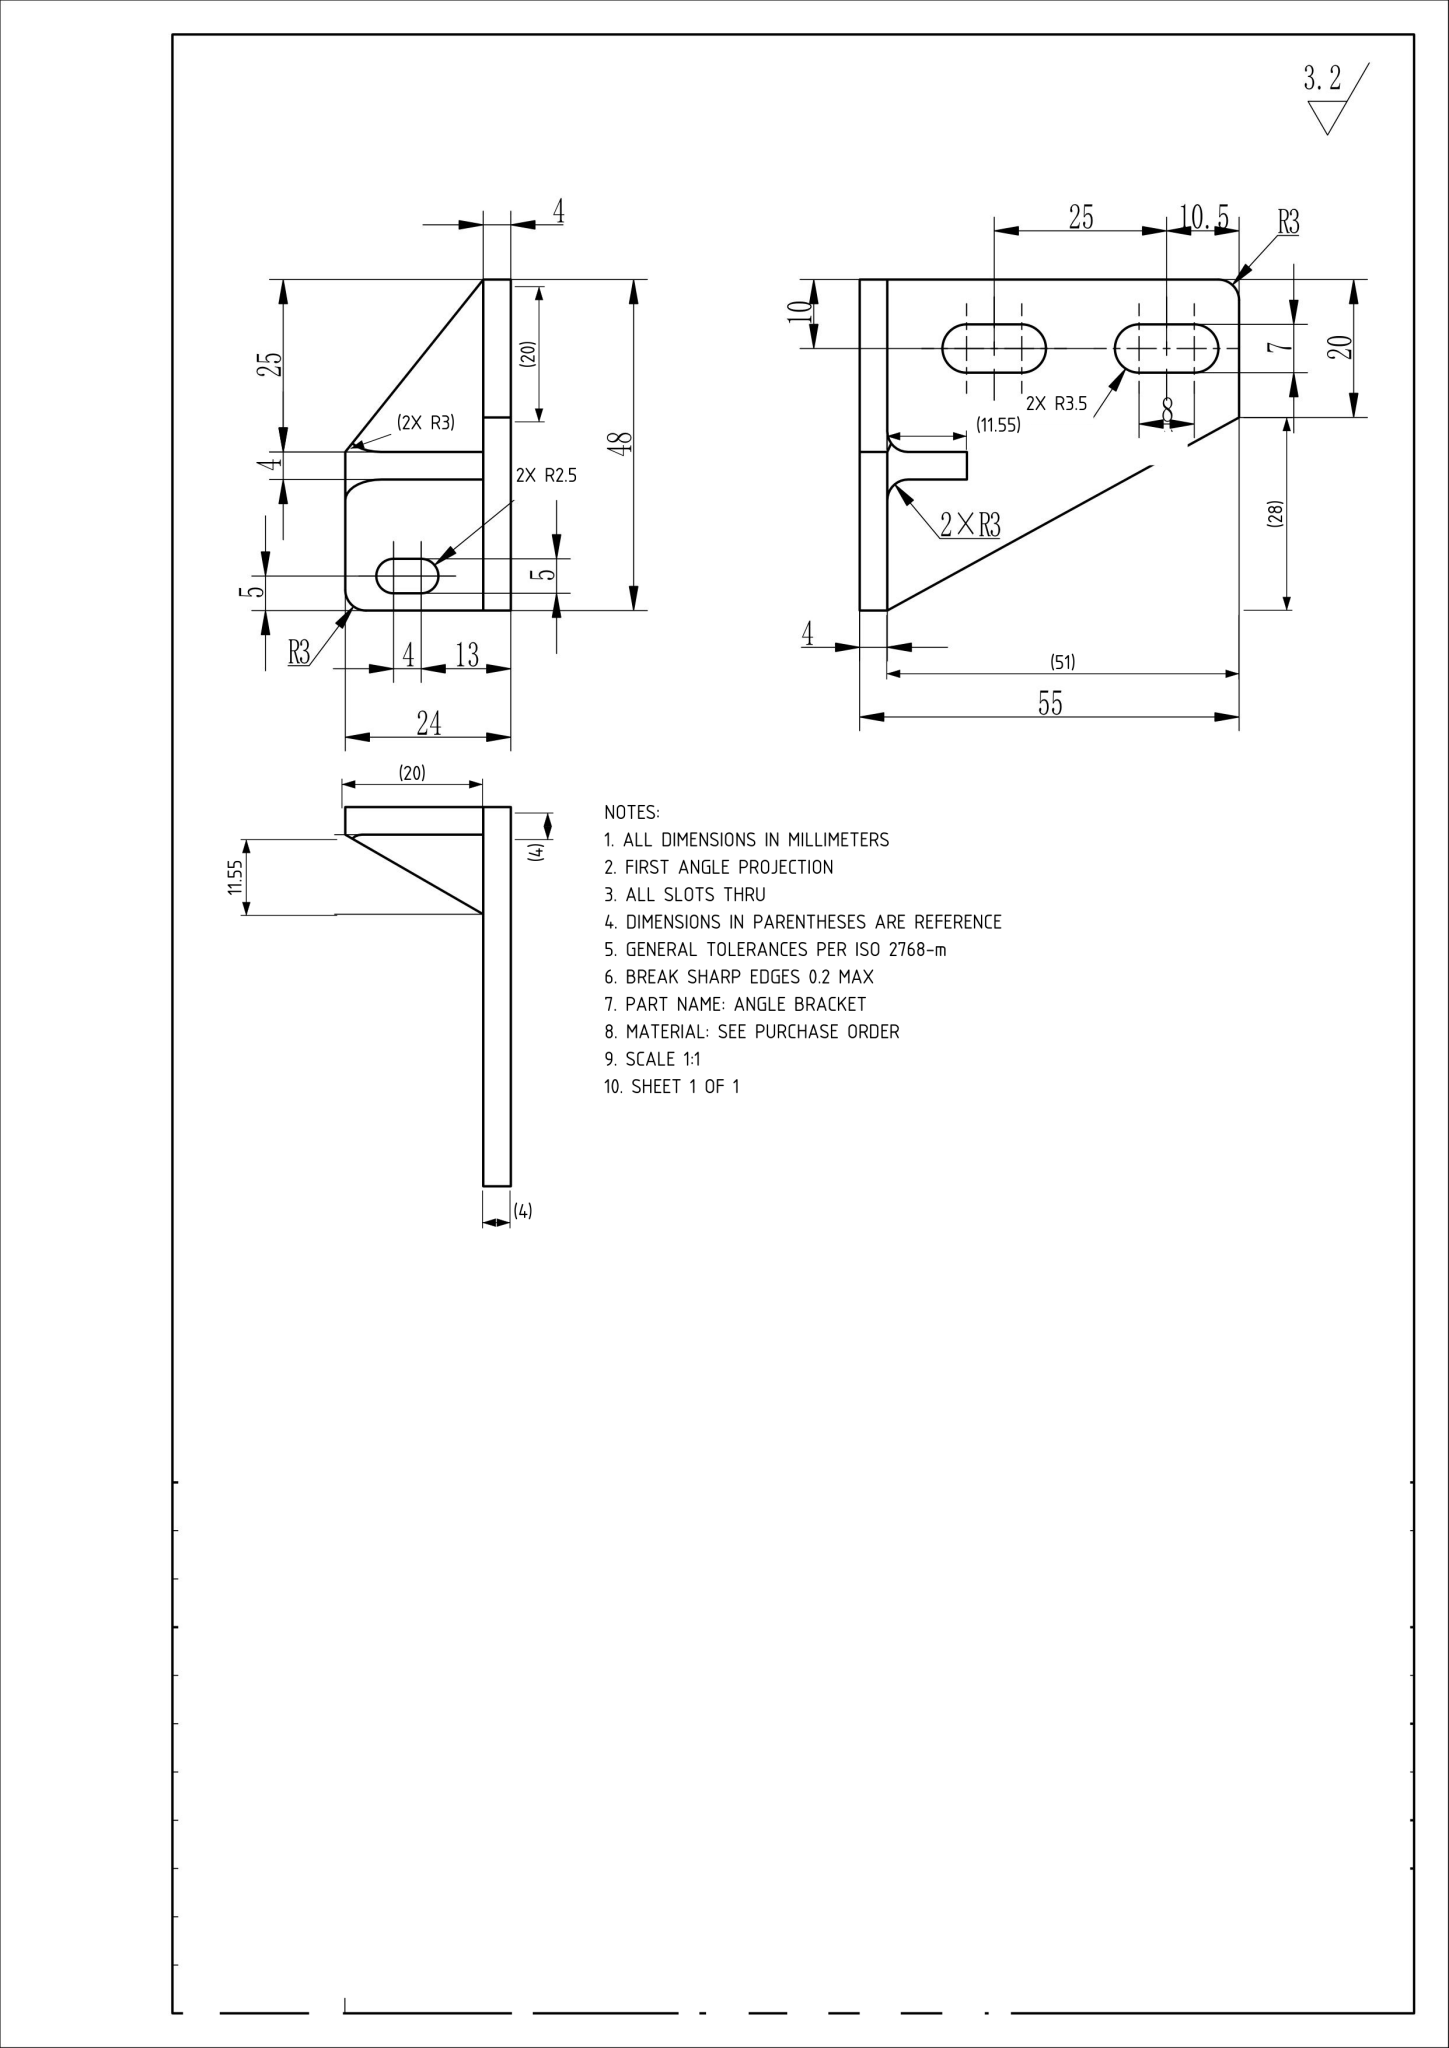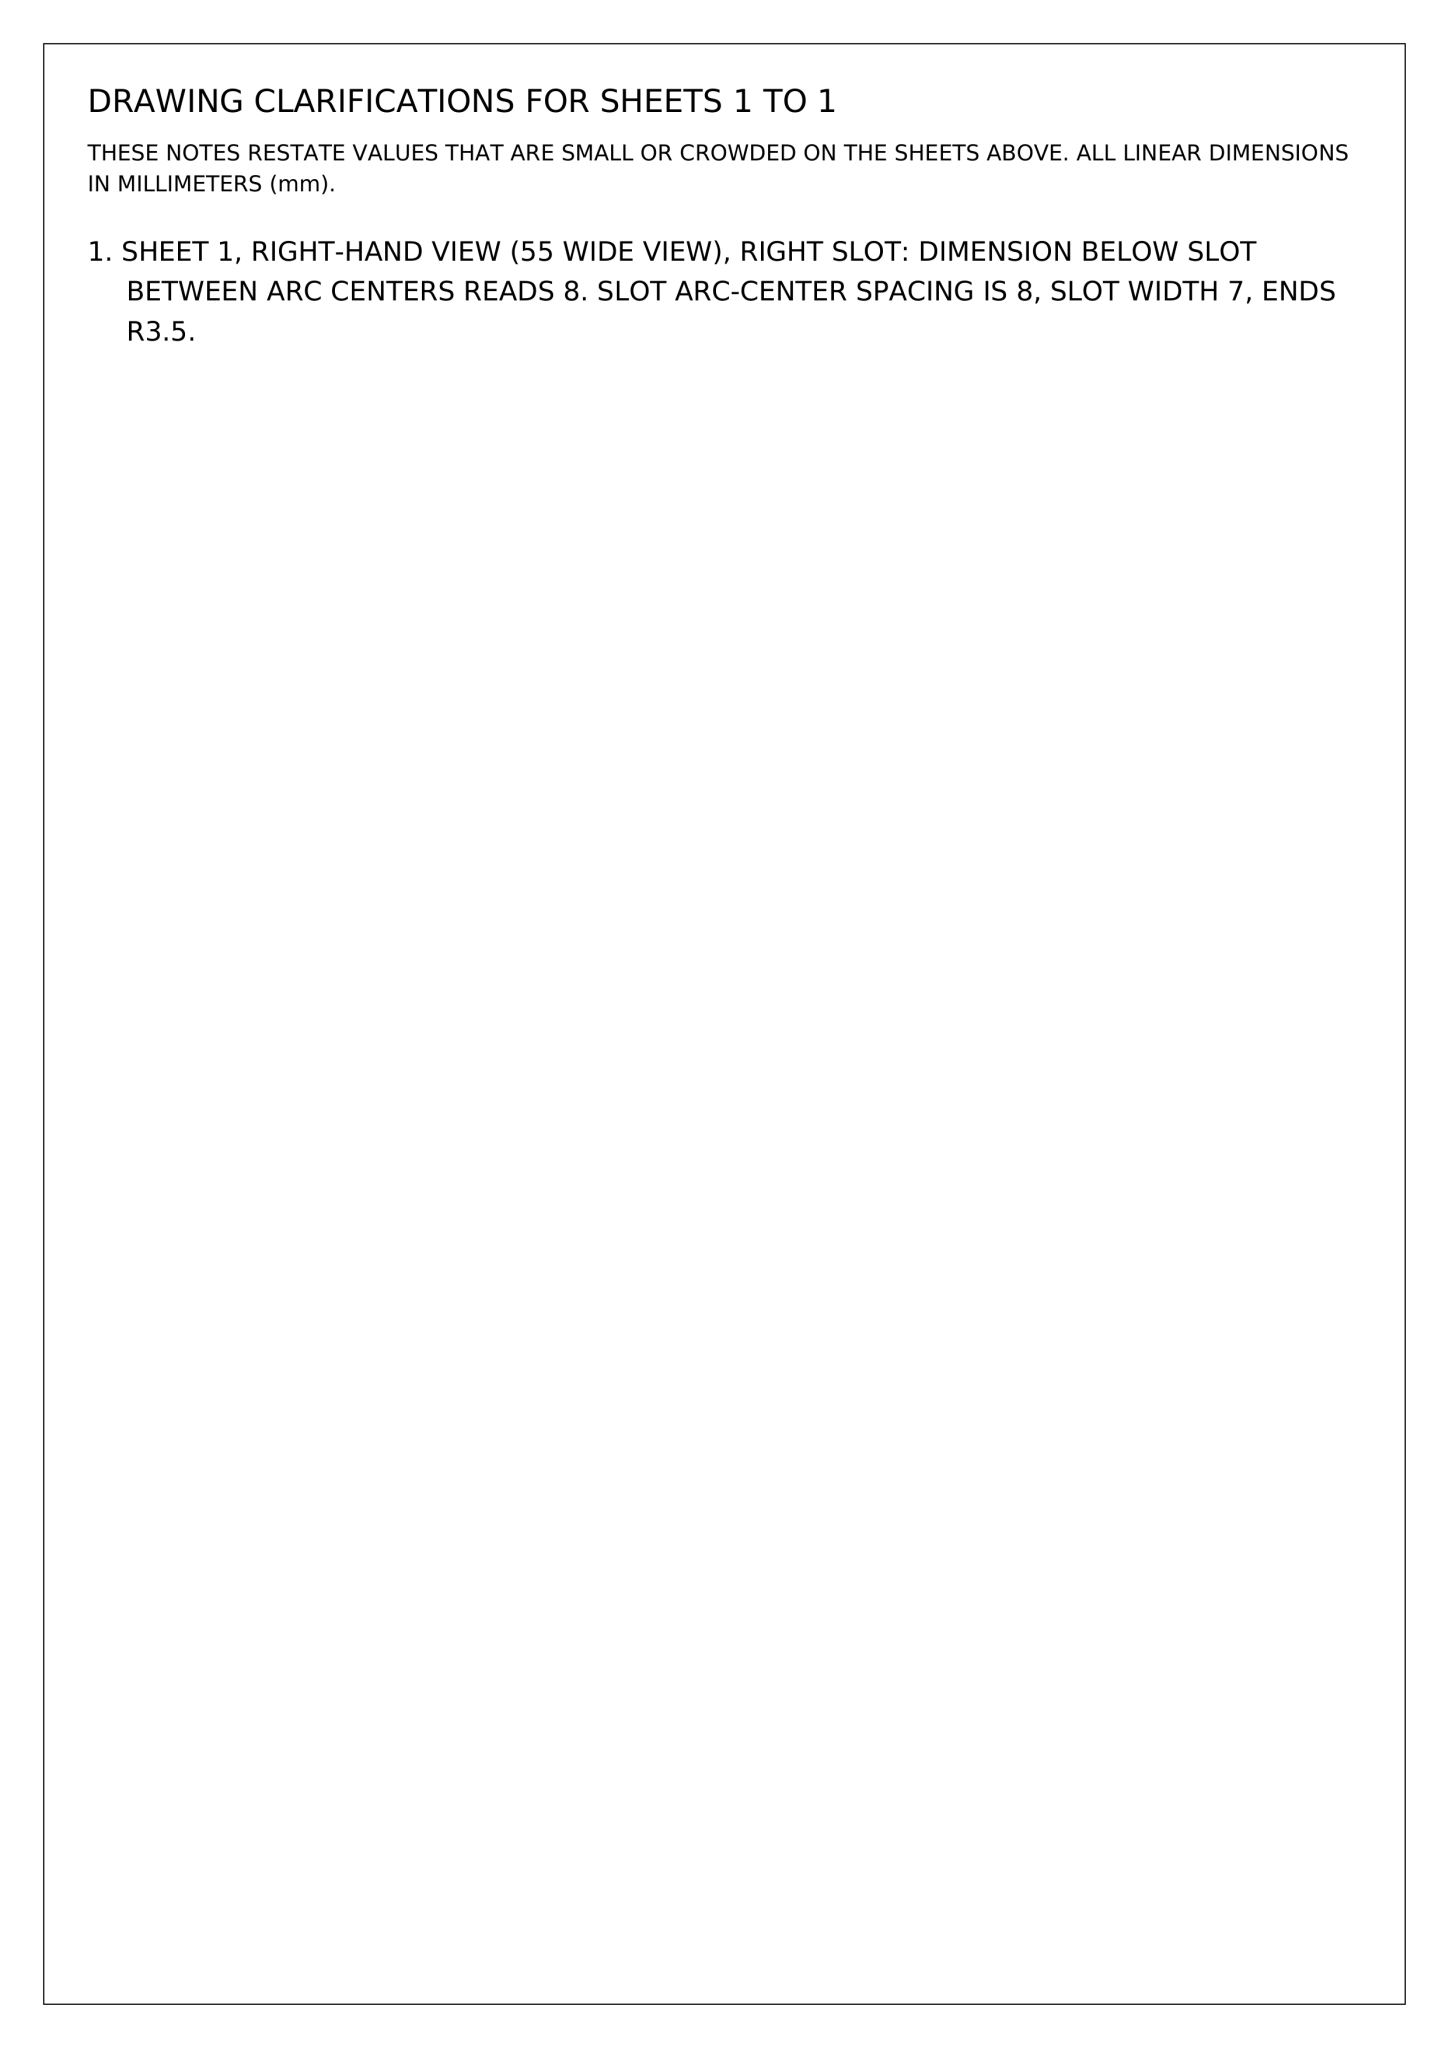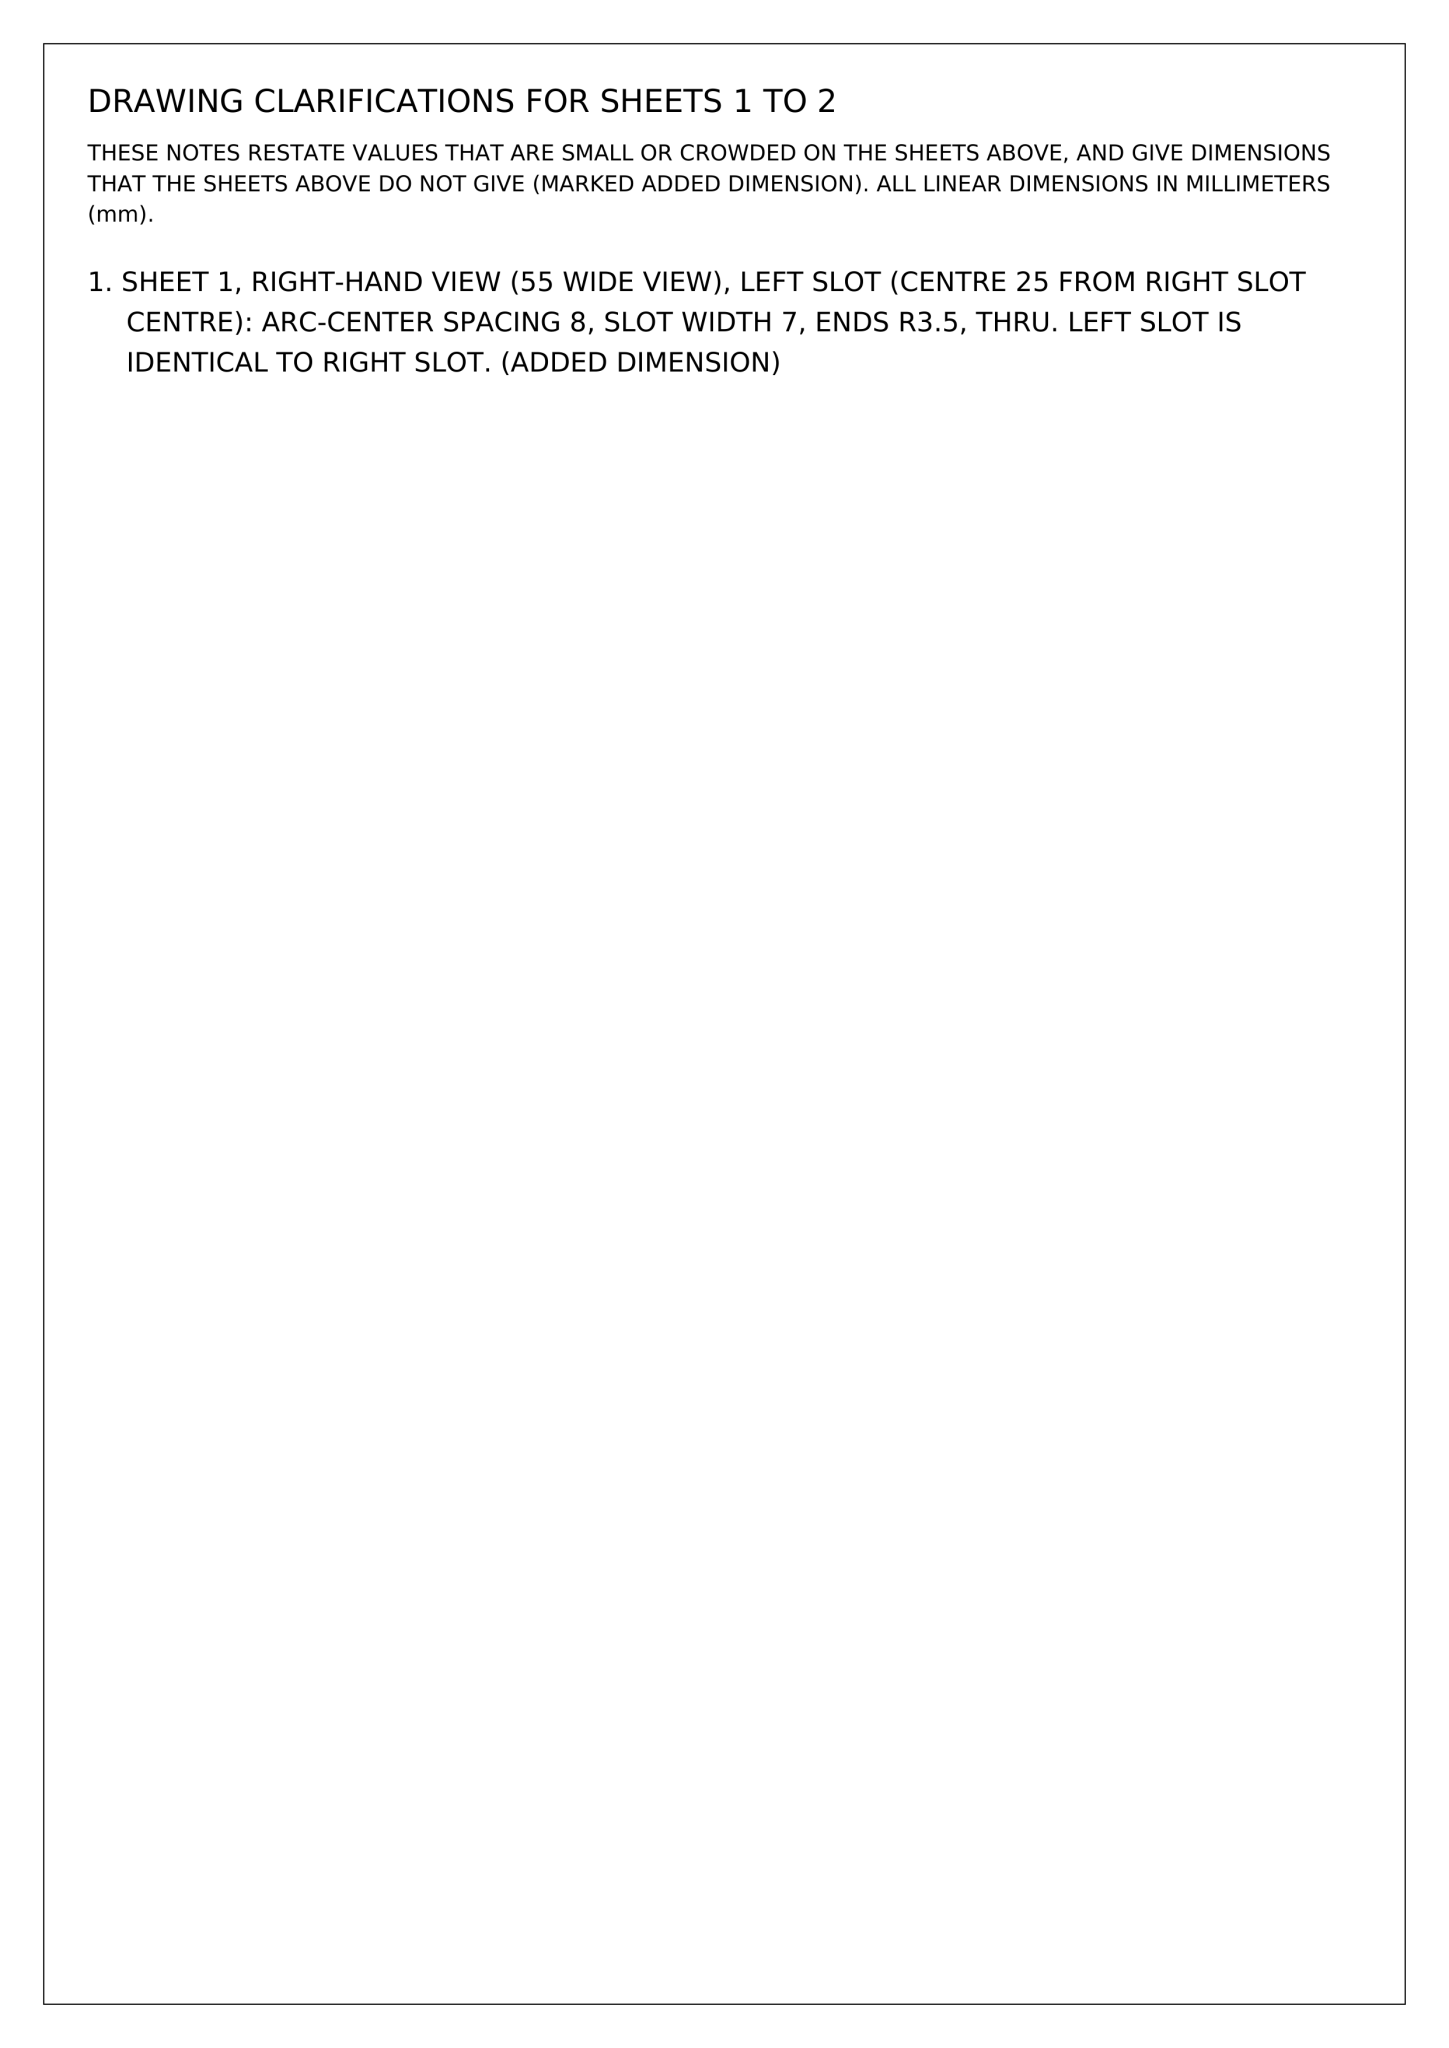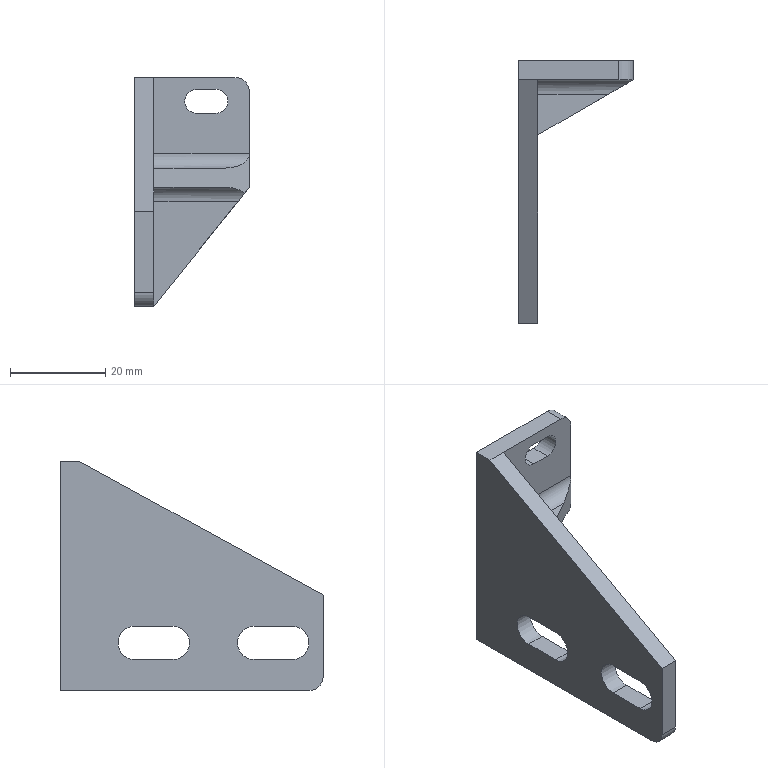Part | NX | mm | 1 solid | 30 faces | box 24 x 55 x 48 mm | volume 10148 mm3 | plane 20 | cylinder 10 | commonest cylinder face diameters 7 x4 6 x4 5 x2